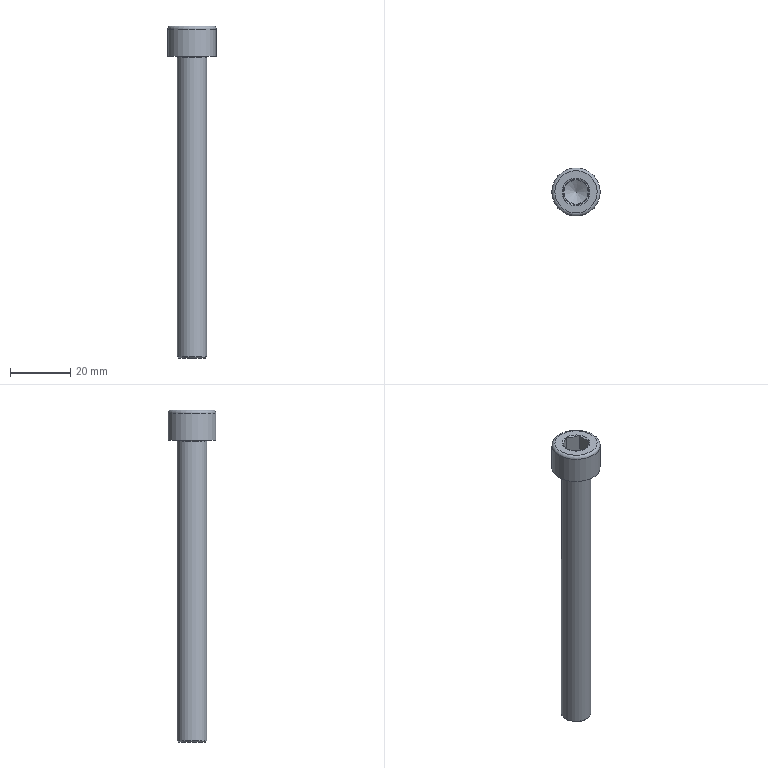Component | NX | GB-T70_1-2000_M10X100_3 | 1 solid | 27 faces | volume 9063 mm3 | plane 15 | cone 8 | cylinder 2 | torus 2 | commonest cylinder face diameters 9.732 x1 16 x1